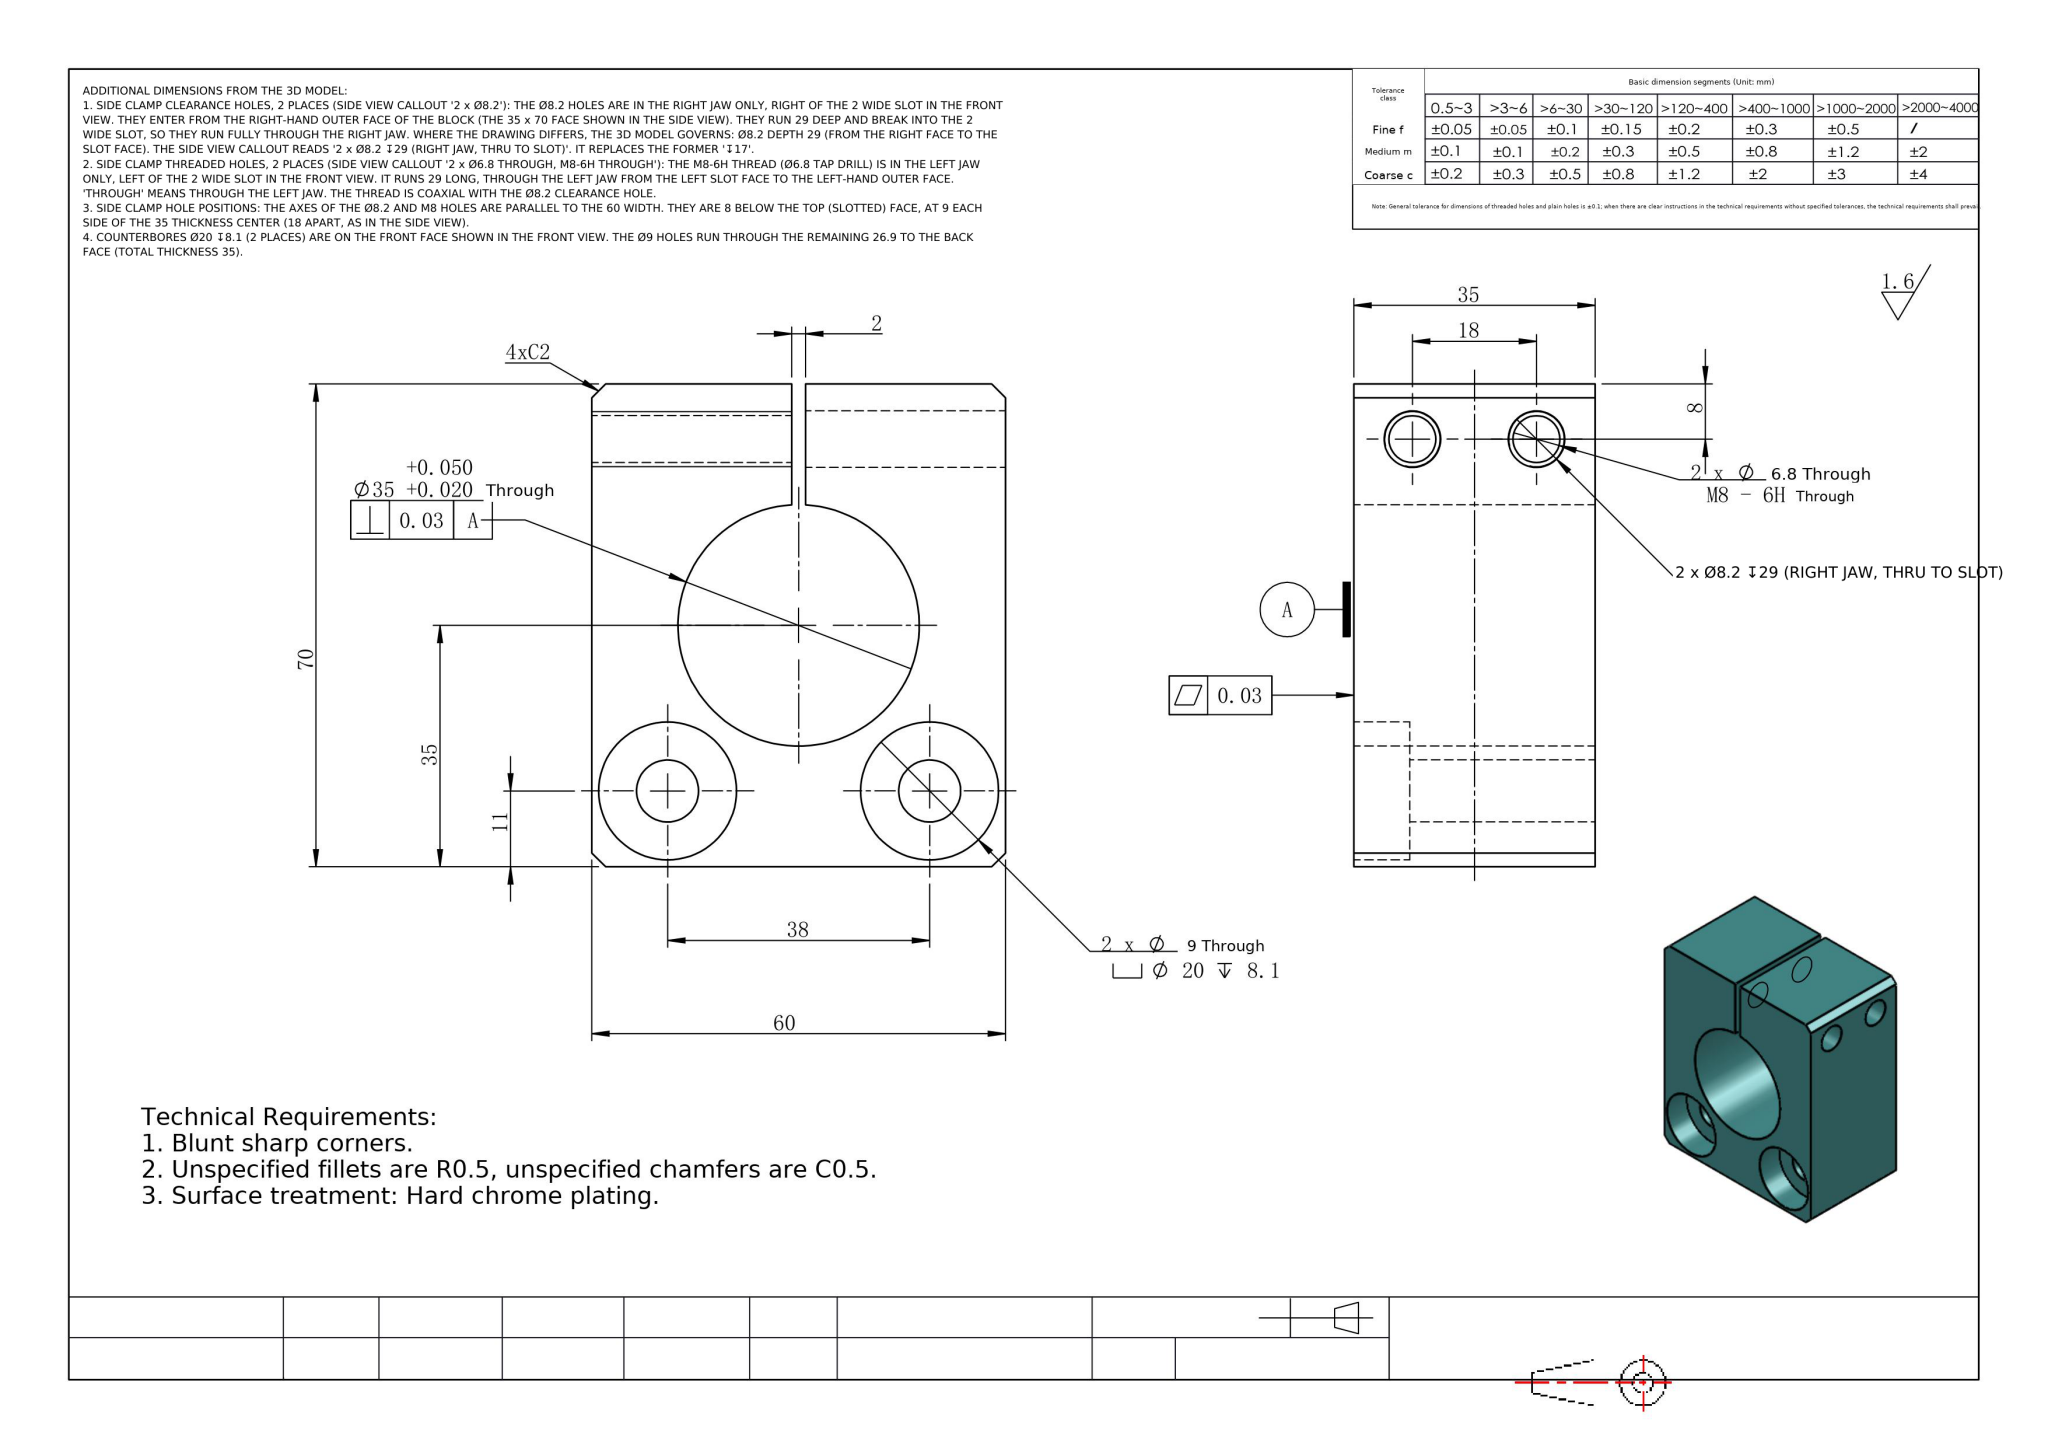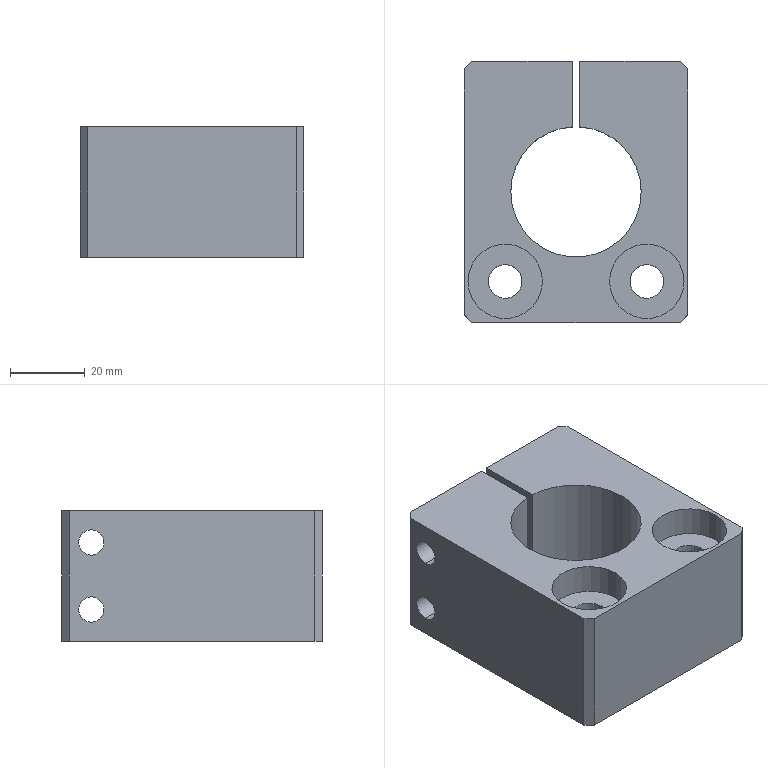Part | NX | mm | Stepped Multi-Bore Cylindrical Cutout Mounting Block | 1 solid | 34 faces | box 60 x 70 x 35 mm | volume 98139 mm3 | cylinder 19 | plane 15 | commonest cylinder face diameters 20 x4 9 x4 6.8 x4 8.2 x4 35 x3